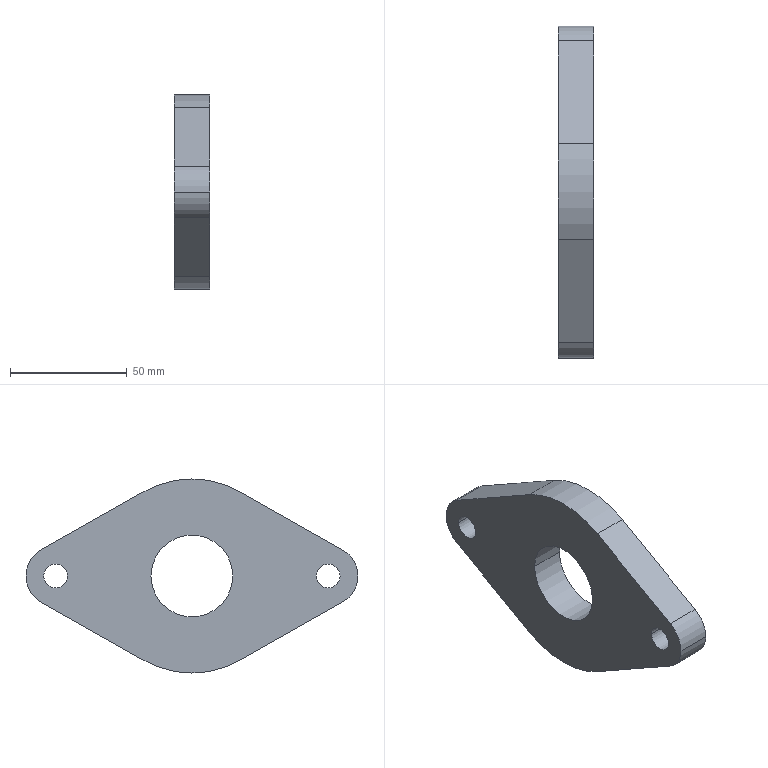Component | SolidWorks | BearingBasePlate-1 | 1 solid | 17 faces | box 15 x 142 x 83 mm | volume 97380 mm3 | cylinder 11 | plane 6 | commonest cylinder face diameters 10.2 x4 25.5 x3 35 x2 83 x2
build123d program:
from build123d import *

# Parameters (mm, degrees)
SKETCH1_R           = 17.5
BOSS_EXTRUDE1_DEPTH = 15
M12_TAPPED_HOLE1_D  = 10.2


with BuildPart() as part:
    # Sketch1 → Boss-Extrude1 (new body)
    with BuildSketch(Plane.XY):
        with BuildLine():
            Line((-20.483, 36.093), (-64.543, 11.089))
            ThreePointArc((-64.543, 11.089), (-71, 0), (-64.543, -11.089))
            Line((-64.543, -11.089), (-20.483, -36.093))
            ThreePointArc((-20.483, -36.093), (0, -41.5), (20.483, -36.093))
            Line((20.483, -36.093), (64.543, -11.089))
            ThreePointArc((64.543, -11.089), (71, 0), (64.543, 11.089))
            Line((64.543, 11.089), (20.483, 36.093))
            ThreePointArc((20.483, 36.093), (0, 41.5), (-20.483, 36.093))
        make_face()
        Circle(SKETCH1_R, mode=Mode.SUBTRACT)
    extrude(amount=BOSS_EXTRUDE1_DEPTH)

    # M12 Tapped Hole1 (through all)
    with Locations(Plane(origin=(0, 0, 0), x_dir=(-1, 0, 0), z_dir=(0, 0, -1))):
        with Locations((-58.25, 0), (58.25, 0)):
            Hole(M12_TAPPED_HOLE1_D / 2)


solid = part.part

# Placed as in the assembly
solid = solid.moved(Location((409.468, 364.666, 811.399), (90, -90, 0)))
STEP:
#1=CARTESIAN_POINT('',(15.53,16.851,31.945));
#2=VERTEX_POINT('',#1);
#3=CARTESIAN_POINT('',(15.53,16.449,31.945));
#4=VERTEX_POINT('',#3);
#5=CARTESIAN_POINT('',(15.53,16.65,31.945));
#6=DIRECTION('',(1.,0.,-0.));
#7=DIRECTION('',(0.,-1.,0.));
#8=AXIS2_PLACEMENT_3D('',#5,#6,#7);
#9=CIRCLE('',#8,0.2008);
#10=EDGE_CURVE('',#2,#4,#9,.T.);
#11=ORIENTED_EDGE('',*,*,#10,.F.);
#12=CARTESIAN_POINT('',(16.121,16.851,31.945));
#13=VERTEX_POINT('',#12);
#14=CARTESIAN_POINT('',(16.121,16.851,31.945));
#15=DIRECTION('',(1.,0.,-0.));
#16=VECTOR('',#15,39.37);
#17=LINE('',#14,#16);
#18=EDGE_CURVE('',#2,#13,#17,.T.);
#19=ORIENTED_EDGE('',*,*,#18,.T.);
#20=CARTESIAN_POINT('',(16.121,16.449,31.945));
#21=VERTEX_POINT('',#20);
#22=CARTESIAN_POINT('',(16.121,16.65,31.945));
#23=DIRECTION('',(1.,0.,-0.));
#24=DIRECTION('',(0.,-1.,0.));
#25=AXIS2_PLACEMENT_3D('',#22,#23,#24);
#26=CIRCLE('',#25,0.2008);
#27=EDGE_CURVE('',#13,#21,#26,.T.);
#28=ORIENTED_EDGE('',*,*,#27,.T.);
#29=CARTESIAN_POINT('',(16.121,16.449,31.945));
#30=DIRECTION('',(1.,0.,-0.));
#31=VECTOR('',#30,39.37);
#32=LINE('',#29,#31);
#33=EDGE_CURVE('',#4,#21,#32,.T.);
#34=ORIENTED_EDGE('',*,*,#33,.F.);
#35=EDGE_LOOP('',(#11,#19,#28,#34));
#36=FACE_OUTER_BOUND('',#35,.T.);
#37=CARTESIAN_POINT('',(16.121,16.65,31.945));
#38=DIRECTION('',(1.,0.,-0.));
#39=DIRECTION('',(0.,-1.,0.));
#40=AXIS2_PLACEMENT_3D('',#37,#38,#39);
#41=CYLINDRICAL_SURFACE('',#40,0.2008);
#42=ADVANCED_FACE('',(#36),#41,.F.);
#43=CARTESIAN_POINT('',(15.53,12.264,31.945));
#44=VERTEX_POINT('',#43);
#45=CARTESIAN_POINT('',(15.53,11.863,31.945));
#46=VERTEX_POINT('',#45);
#47=CARTESIAN_POINT('',(15.53,12.064,31.945));
#48=DIRECTION('',(1.,0.,-0.));
#49=DIRECTION('',(0.,-1.,0.));
#50=AXIS2_PLACEMENT_3D('',#47,#48,#49);
#51=CIRCLE('',#50,0.2008);
#52=EDGE_CURVE('',#44,#46,#51,.T.);
#53=ORIENTED_EDGE('',*,*,#52,.F.);
#54=CARTESIAN_POINT('',(16.121,12.264,31.945));
#55=VERTEX_POINT('',#54);
#56=CARTESIAN_POINT('',(16.121,12.264,31.945));
#57=DIRECTION('',(1.,0.,-0.));
#58=VECTOR('',#57,39.37);
#59=LINE('',#56,#58);
#60=EDGE_CURVE('',#44,#55,#59,.T.);
#61=ORIENTED_EDGE('',*,*,#60,.T.);
#62=CARTESIAN_POINT('',(16.121,11.863,31.945));
#63=VERTEX_POINT('',#62);
#64=CARTESIAN_POINT('',(16.121,12.064,31.945));
#65=DIRECTION('',(1.,0.,-0.));
#66=DIRECTION('',(0.,-1.,0.));
#67=AXIS2_PLACEMENT_3D('',#64,#65,#66);
#68=CIRCLE('',#67,0.2008);
#69=EDGE_CURVE('',#55,#63,#68,.T.);
#70=ORIENTED_EDGE('',*,*,#69,.T.);
#71=CARTESIAN_POINT('',(16.121,11.863,31.945));
#72=DIRECTION('',(1.,0.,-0.));
#73=VECTOR('',#72,39.37);
#74=LINE('',#71,#73);
#75=EDGE_CURVE('',#46,#63,#74,.T.);
#76=ORIENTED_EDGE('',*,*,#75,.F.);
#77=EDGE_LOOP('',(#53,#61,#70,#76));
#78=FACE_OUTER_BOUND('',#77,.T.);
#79=CARTESIAN_POINT('',(16.121,12.064,31.945));
#80=DIRECTION('',(1.,0.,-0.));
#81=DIRECTION('',(0.,-1.,0.));
#82=AXIS2_PLACEMENT_3D('',#79,#80,#81);
#83=CYLINDRICAL_SURFACE('',#82,0.2008);
#84=ADVANCED_FACE('',(#78),#83,.F.);
#85=CARTESIAN_POINT('',(15.53,13.668,31.945));
#86=VERTEX_POINT('',#85);
#87=CARTESIAN_POINT('',(15.53,15.046,31.945));
#88=VERTEX_POINT('',#87);
#89=CARTESIAN_POINT('',(15.53,14.357,31.945));
#90=DIRECTION('',(-1.,-0.,0.));
#91=DIRECTION('',(0.,1.,0.));
#92=AXIS2_PLACEMENT_3D('',#89,#90,#91);
#93=CIRCLE('',#92,0.689);
#94=EDGE_CURVE('',#86,#88,#93,.T.);
#95=ORIENTED_EDGE('',*,*,#94,.T.);
#96=CARTESIAN_POINT('',(16.121,15.046,31.945));
#97=VERTEX_POINT('',#96);
#98=CARTESIAN_POINT('',(15.53,15.046,31.945));
#99=DIRECTION('',(1.,0.,-0.));
#100=VECTOR('',#99,39.37);
#101=LINE('',#98,#100);
#102=EDGE_CURVE('',#88,#97,#101,.T.);
#103=ORIENTED_EDGE('',*,*,#102,.T.);
#104=CARTESIAN_POINT('',(16.121,13.668,31.945));
#105=VERTEX_POINT('',#104);
#106=CARTESIAN_POINT('',(16.121,14.357,31.945));
#107=DIRECTION('',(-1.,-0.,0.));
#108=DIRECTION('',(0.,1.,0.));
#109=AXIS2_PLACEMENT_3D('',#106,#107,#108);
#110=CIRCLE('',#109,0.689);
#111=EDGE_CURVE('',#105,#97,#110,.T.);
#112=ORIENTED_EDGE('',*,*,#111,.F.);
#113=CARTESIAN_POINT('',(15.53,13.668,31.945));
#114=DIRECTION('',(1.,0.,-0.));
#115=VECTOR('',#114,39.37);
#116=LINE('',#113,#115);
#117=EDGE_CURVE('',#86,#105,#116,.T.);
#118=ORIENTED_EDGE('',*,*,#117,.F.);
#119=EDGE_LOOP('',(#95,#103,#112,#118));
#120=FACE_OUTER_BOUND('',#119,.T.);
#121=CARTESIAN_POINT('',(15.53,14.357,31.945));
#122=DIRECTION('',(1.,0.,-0.));
#123=DIRECTION('',(0.,-1.,0.));
#124=AXIS2_PLACEMENT_3D('',#121,#122,#123);
#125=CYLINDRICAL_SURFACE('',#124,0.689);
#126=ADVANCED_FACE('',(#120),#125,.F.);
#127=CARTESIAN_POINT('',(15.53,11.562,31.945));
#128=VERTEX_POINT('',#127);
#129=CARTESIAN_POINT('',(15.53,11.816,32.381));
#130=VERTEX_POINT('',#129);
#131=CARTESIAN_POINT('',(15.53,12.064,31.945));
#132=DIRECTION('',(-1.,-0.,0.));
#133=DIRECTION('',(0.,1.,0.));
#134=AXIS2_PLACEMENT_3D('',#131,#132,#133);
#135=CIRCLE('',#134,0.502);
#136=EDGE_CURVE('',#128,#130,#135,.T.);
#137=ORIENTED_EDGE('',*,*,#136,.F.);
#138=CARTESIAN_POINT('',(16.121,11.562,31.945));
#139=VERTEX_POINT('',#138);
#140=CARTESIAN_POINT('',(15.53,11.562,31.945));
#141=DIRECTION('',(1.,0.,-0.));
#142=VECTOR('',#141,39.37);
#143=LINE('',#140,#142);
#144=EDGE_CURVE('',#128,#139,#143,.T.);
#145=ORIENTED_EDGE('',*,*,#144,.T.);
#146=CARTESIAN_POINT('',(16.121,11.816,32.381));
#147=VERTEX_POINT('',#146);
#148=CARTESIAN_POINT('',(16.121,12.064,31.945));
#149=DIRECTION('',(-1.,-0.,0.));
#150=DIRECTION('',(0.,1.,0.));
#151=AXIS2_PLACEMENT_3D('',#148,#149,#150);
#152=CIRCLE('',#151,0.502);
#153=EDGE_CURVE('',#139,#147,#152,.T.);
#154=ORIENTED_EDGE('',*,*,#153,.T.);
#155=CARTESIAN_POINT('',(15.53,11.816,32.381));
#156=DIRECTION('',(1.,0.,-0.));
#157=VECTOR('',#156,39.37);
#158=LINE('',#155,#157);
#159=EDGE_CURVE('',#130,#147,#158,.T.);
#160=ORIENTED_EDGE('',*,*,#159,.F.);
#161=EDGE_LOOP('',(#137,#145,#154,#160));
#162=FACE_OUTER_BOUND('',#161,.T.);
#163=CARTESIAN_POINT('',(15.53,12.064,31.945));
#164=DIRECTION('',(1.,0.,-0.));
#165=DIRECTION('',(0.,-1.,0.));
#166=AXIS2_PLACEMENT_3D('',#163,#164,#165);
#167=CYLINDRICAL_SURFACE('',#166,0.502);
#168=ADVANCED_FACE('',(#162),#167,.T.);
#169=CARTESIAN_POINT('',(15.53,16.65,31.945));
#170=DIRECTION('',(1.,0.,-0.));
#171=DIRECTION('',(0.,-1.,0.));
#172=AXIS2_PLACEMENT_3D('',#169,#170,#171);
#173=CIRCLE('',#172,0.2008);
#174=EDGE_CURVE('',#4,#2,#173,.T.);
#175=ORIENTED_EDGE('',*,*,#174,.T.);
#176=ORIENTED_EDGE('',*,*,#10,.T.);
#177=EDGE_LOOP('',(#175,#176));
#178=FACE_BOUND('',#177,.T.);
#179=CARTESIAN_POINT('',(15.53,12.064,31.945));
#180=DIRECTION('',(1.,0.,-0.));
#181=DIRECTION('',(0.,-1.,0.));
#182=AXIS2_PLACEMENT_3D('',#179,#180,#181);
#183=CIRCLE('',#182,0.2008);
#184=EDGE_CURVE('',#46,#44,#183,.T.);
#185=ORIENTED_EDGE('',*,*,#184,.T.);
#186=ORIENTED_EDGE('',*,*,#52,.T.);
#187=EDGE_LOOP('',(#185,#186));
#188=FACE_BOUND('',#187,.T.);
#189=CARTESIAN_POINT('',(15.53,15.163,30.524));
#190=VERTEX_POINT('',#189);
#191=CARTESIAN_POINT('',(15.53,13.551,30.524));
#192=VERTEX_POINT('',#191);
#193=CARTESIAN_POINT('',(15.53,14.357,31.945));
#194=DIRECTION('',(-1.,-0.,0.));
#195=DIRECTION('',(0.,1.,0.));
#196=AXIS2_PLACEMENT_3D('',#193,#194,#195);
#197=CIRCLE('',#196,1.634);
#198=EDGE_CURVE('',#190,#192,#197,.T.);
#199=ORIENTED_EDGE('',*,*,#198,.T.);
#200=CARTESIAN_POINT('',(15.53,11.816,31.508));
#201=VERTEX_POINT('',#200);
#202=CARTESIAN_POINT('',(15.53,13.551,30.524));
#203=DIRECTION('',(0.,-0.8697,0.4936));
#204=VECTOR('',#203,39.37);
#205=LINE('',#202,#204);
#206=EDGE_CURVE('',#192,#201,#205,.T.);
#207=ORIENTED_EDGE('',*,*,#206,.T.);
#208=CARTESIAN_POINT('',(15.53,12.064,31.945));
#209=DIRECTION('',(-1.,-0.,0.));
#210=DIRECTION('',(0.,1.,0.));
#211=AXIS2_PLACEMENT_3D('',#208,#209,#210);
#212=CIRCLE('',#211,0.502);
#213=EDGE_CURVE('',#201,#128,#212,.T.);
#214=ORIENTED_EDGE('',*,*,#213,.T.);
#215=ORIENTED_EDGE('',*,*,#136,.T.);
#216=CARTESIAN_POINT('',(15.53,13.551,33.366));
#217=VERTEX_POINT('',#216);
#218=CARTESIAN_POINT('',(15.53,11.816,32.381));
#219=DIRECTION('',(0.,0.8697,0.4936));
#220=VECTOR('',#219,39.37);
#221=LINE('',#218,#220);
#222=EDGE_CURVE('',#130,#217,#221,.T.);
#223=ORIENTED_EDGE('',*,*,#222,.T.);
#224=CARTESIAN_POINT('',(15.53,15.163,33.366));
#225=VERTEX_POINT('',#224);
#226=CARTESIAN_POINT('',(15.53,14.357,31.945));
#227=DIRECTION('',(-1.,-0.,0.));
#228=DIRECTION('',(0.,1.,0.));
#229=AXIS2_PLACEMENT_3D('',#226,#227,#228);
#230=CIRCLE('',#229,1.634);
#231=EDGE_CURVE('',#217,#225,#230,.T.);
#232=ORIENTED_EDGE('',*,*,#231,.T.);
#233=CARTESIAN_POINT('',(15.53,16.898,32.381));
#234=VERTEX_POINT('',#233);
#235=CARTESIAN_POINT('',(15.53,15.163,33.366));
#236=DIRECTION('',(-0.,0.8697,-0.4936));
#237=VECTOR('',#236,39.37);
#238=LINE('',#235,#237);
#239=EDGE_CURVE('',#225,#234,#238,.T.);
#240=ORIENTED_EDGE('',*,*,#239,.T.);
#241=CARTESIAN_POINT('',(15.53,16.898,31.508));
#242=VERTEX_POINT('',#241);
#243=CARTESIAN_POINT('',(15.53,16.65,31.945));
#244=DIRECTION('',(-1.,-0.,0.));
#245=DIRECTION('',(0.,1.,0.));
#246=AXIS2_PLACEMENT_3D('',#243,#244,#245);
#247=CIRCLE('',#246,0.502);
#248=EDGE_CURVE('',#234,#242,#247,.T.);
#249=ORIENTED_EDGE('',*,*,#248,.T.);
#250=CARTESIAN_POINT('',(15.53,16.898,31.508));
#251=DIRECTION('',(-0.,-0.8697,-0.4936));
#252=VECTOR('',#251,39.37);
#253=LINE('',#250,#252);
#254=EDGE_CURVE('',#242,#190,#253,.T.);
#255=ORIENTED_EDGE('',*,*,#254,.T.);
#256=EDGE_LOOP('',(#199,#207,#214,#215,#223,#232,#240,#249,#255));
#257=FACE_OUTER_BOUND('',#256,.T.);
#258=ORIENTED_EDGE('',*,*,#94,.F.);
#259=CARTESIAN_POINT('',(15.53,14.357,31.945));
#260=DIRECTION('',(-1.,-0.,0.));
#261=DIRECTION('',(0.,1.,0.));
#262=AXIS2_PLACEMENT_3D('',#259,#260,#261);
#263=CIRCLE('',#262,0.689);
#264=EDGE_CURVE('',#88,#86,#263,.T.);
#265=ORIENTED_EDGE('',*,*,#264,.F.);
#266=EDGE_LOOP('',(#258,#265));
#267=FACE_BOUND('',#266,.T.);
#268=CARTESIAN_POINT('',(15.53,14.357,31.945));
#269=DIRECTION('',(-1.,-0.,0.));
#270=DIRECTION('',(-0.,1.,0.));
#271=AXIS2_PLACEMENT_3D('',#268,#269,#270);
#272=PLANE('',#271);
#273=ADVANCED_FACE('',(#178,#188,#257,#267),#272,.T.);
#274=CARTESIAN_POINT('',(16.121,16.65,31.945));
#275=DIRECTION('',(1.,0.,-0.));
#276=DIRECTION('',(0.,-1.,0.));
#277=AXIS2_PLACEMENT_3D('',#274,#275,#276);
#278=CIRCLE('',#277,0.2008);
#279=EDGE_CURVE('',#21,#13,#278,.T.);
#280=ORIENTED_EDGE('',*,*,#279,.F.);
#281=ORIENTED_EDGE('',*,*,#27,.F.);
#282=EDGE_LOOP('',(#280,#281));
#283=FACE_BOUND('',#282,.T.);
#284=CARTESIAN_POINT('',(16.121,12.064,31.945));
#285=DIRECTION('',(1.,0.,-0.));
#286=DIRECTION('',(0.,-1.,0.));
#287=AXIS2_PLACEMENT_3D('',#284,#285,#286);
#288=CIRCLE('',#287,0.2008);
#289=EDGE_CURVE('',#63,#55,#288,.T.);
#290=ORIENTED_EDGE('',*,*,#289,.F.);
#291=ORIENTED_EDGE('',*,*,#69,.F.);
#292=EDGE_LOOP('',(#290,#291));
#293=FACE_BOUND('',#292,.T.);
#294=CARTESIAN_POINT('',(16.121,15.163,30.524));
#295=VERTEX_POINT('',#294);
#296=CARTESIAN_POINT('',(16.121,13.551,30.524));
#297=VERTEX_POINT('',#296);
#298=CARTESIAN_POINT('',(16.121,14.357,31.945));
#299=DIRECTION('',(-1.,-0.,0.));
#300=DIRECTION('',(0.,1.,0.));
#301=AXIS2_PLACEMENT_3D('',#298,#299,#300);
#302=CIRCLE('',#301,1.634);
#303=EDGE_CURVE('',#295,#297,#302,.T.);
#304=ORIENTED_EDGE('',*,*,#303,.F.);
#305=CARTESIAN_POINT('',(16.121,16.898,31.508));
#306=VERTEX_POINT('',#305);
#307=CARTESIAN_POINT('',(16.121,16.898,31.508));
#308=DIRECTION('',(-0.,-0.8697,-0.4936));
#309=VECTOR('',#308,39.37);
#310=LINE('',#307,#309);
#311=EDGE_CURVE('',#306,#295,#310,.T.);
#312=ORIENTED_EDGE('',*,*,#311,.F.);
#313=CARTESIAN_POINT('',(16.121,16.898,32.381));
#314=VERTEX_POINT('',#313);
#315=CARTESIAN_POINT('',(16.121,16.65,31.945));
#316=DIRECTION('',(-1.,-0.,0.));
#317=DIRECTION('',(0.,1.,0.));
#318=AXIS2_PLACEMENT_3D('',#315,#316,#317);
#319=CIRCLE('',#318,0.502);
#320=EDGE_CURVE('',#314,#306,#319,.T.);
#321=ORIENTED_EDGE('',*,*,#320,.F.);
#322=CARTESIAN_POINT('',(16.121,15.163,33.366));
#323=VERTEX_POINT('',#322);
#324=CARTESIAN_POINT('',(16.121,15.163,33.366));
#325=DIRECTION('',(-0.,0.8697,-0.4936));
#326=VECTOR('',#325,39.37);
#327=LINE('',#324,#326);
#328=EDGE_CURVE('',#323,#314,#327,.T.);
#329=ORIENTED_EDGE('',*,*,#328,.F.);
#330=CARTESIAN_POINT('',(16.121,13.551,33.366));
#331=VERTEX_POINT('',#330);
#332=CARTESIAN_POINT('',(16.121,14.357,31.945));
#333=DIRECTION('',(-1.,-0.,0.));
#334=DIRECTION('',(0.,1.,0.));
#335=AXIS2_PLACEMENT_3D('',#332,#333,#334);
#336=CIRCLE('',#335,1.634);
#337=EDGE_CURVE('',#331,#323,#336,.T.);
#338=ORIENTED_EDGE('',*,*,#337,.F.);
#339=CARTESIAN_POINT('',(16.121,11.816,32.381));
#340=DIRECTION('',(0.,0.8697,0.4936));
#341=VECTOR('',#340,39.37);
#342=LINE('',#339,#341);
#343=EDGE_CURVE('',#147,#331,#342,.T.);
#344=ORIENTED_EDGE('',*,*,#343,.F.);
#345=ORIENTED_EDGE('',*,*,#153,.F.);
#346=CARTESIAN_POINT('',(16.121,11.816,31.508));
#347=VERTEX_POINT('',#346);
#348=CARTESIAN_POINT('',(16.121,12.064,31.945));
#349=DIRECTION('',(-1.,-0.,0.));
#350=DIRECTION('',(0.,1.,0.));
#351=AXIS2_PLACEMENT_3D('',#348,#349,#350);
#352=CIRCLE('',#351,0.502);
#353=EDGE_CURVE('',#347,#139,#352,.T.);
#354=ORIENTED_EDGE('',*,*,#353,.F.);
#355=CARTESIAN_POINT('',(16.121,13.551,30.524));
#356=DIRECTION('',(0.,-0.8697,0.4936));
#357=VECTOR('',#356,39.37);
#358=LINE('',#355,#357);
#359=EDGE_CURVE('',#297,#347,#358,.T.);
#360=ORIENTED_EDGE('',*,*,#359,.F.);
#361=EDGE_LOOP('',(#304,#312,#321,#329,#338,#344,#345,#354,#360));
#362=FACE_OUTER_BOUND('',#361,.T.);
#363=ORIENTED_EDGE('',*,*,#111,.T.);
#364=CARTESIAN_POINT('',(16.121,14.357,31.945));
#365=DIRECTION('',(-1.,-0.,0.));
#366=DIRECTION('',(0.,1.,0.));
#367=AXIS2_PLACEMENT_3D('',#364,#365,#366);
#368=CIRCLE('',#367,0.689);
#369=EDGE_CURVE('',#97,#105,#368,.T.);
#370=ORIENTED_EDGE('',*,*,#369,.T.);
#371=EDGE_LOOP('',(#363,#370));
#372=FACE_BOUND('',#371,.T.);
#373=CARTESIAN_POINT('',(16.121,14.357,31.945));
#374=DIRECTION('',(-1.,-0.,0.));
#375=DIRECTION('',(-0.,1.,0.));
#376=AXIS2_PLACEMENT_3D('',#373,#374,#375);
#377=PLANE('',#376);
#378=ADVANCED_FACE('',(#283,#293,#362,#372),#377,.F.);
#379=ORIENTED_EDGE('',*,*,#303,.T.);
#380=CARTESIAN_POINT('',(15.53,13.551,30.524));
#381=DIRECTION('',(1.,0.,-0.));
#382=VECTOR('',#381,39.37);
#383=LINE('',#380,#382);
#384=EDGE_CURVE('',#192,#297,#383,.T.);
#385=ORIENTED_EDGE('',*,*,#384,.F.);
#386=ORIENTED_EDGE('',*,*,#198,.F.);
#387=CARTESIAN_POINT('',(15.53,15.163,30.524));
#388=DIRECTION('',(1.,0.,-0.));
#389=VECTOR('',#388,39.37);
#390=LINE('',#387,#389);
#391=EDGE_CURVE('',#190,#295,#390,.T.);
#392=ORIENTED_EDGE('',*,*,#391,.T.);
#393=EDGE_LOOP('',(#379,#385,#386,#392));
#394=FACE_OUTER_BOUND('',#393,.T.);
#395=CARTESIAN_POINT('',(15.53,14.357,31.945));
#396=DIRECTION('',(1.,0.,-0.));
#397=DIRECTION('',(0.,-1.,0.));
#398=AXIS2_PLACEMENT_3D('',#395,#396,#397);
#399=CYLINDRICAL_SURFACE('',#398,1.634);
#400=ADVANCED_FACE('',(#394),#399,.T.);
#401=ORIENTED_EDGE('',*,*,#359,.T.);
#402=CARTESIAN_POINT('',(15.53,11.816,31.508));
#403=DIRECTION('',(1.,0.,-0.));
#404=VECTOR('',#403,39.37);
#405=LINE('',#402,#404);
#406=EDGE_CURVE('',#201,#347,#405,.T.);
#407=ORIENTED_EDGE('',*,*,#406,.F.);
#408=ORIENTED_EDGE('',*,*,#206,.F.);
#409=ORIENTED_EDGE('',*,*,#384,.T.);
#410=EDGE_LOOP('',(#401,#407,#408,#409));
#411=FACE_OUTER_BOUND('',#410,.T.);
#412=CARTESIAN_POINT('',(15.53,13.551,30.524));
#413=DIRECTION('',(0.,0.4936,0.8697));
#414=DIRECTION('',(-0.,0.8697,-0.4936));
#415=AXIS2_PLACEMENT_3D('',#412,#413,#414);
#416=PLANE('',#415);
#417=ADVANCED_FACE('',(#411),#416,.F.);
#418=ORIENTED_EDGE('',*,*,#144,.F.);
#419=ORIENTED_EDGE('',*,*,#213,.F.);
#420=ORIENTED_EDGE('',*,*,#406,.T.);
#421=ORIENTED_EDGE('',*,*,#353,.T.);
#422=EDGE_LOOP('',(#418,#419,#420,#421));
#423=FACE_OUTER_BOUND('',#422,.T.);
#424=CARTESIAN_POINT('',(15.53,12.064,31.945));
#425=DIRECTION('',(1.,0.,-0.));
#426=DIRECTION('',(0.,-1.,0.));
#427=AXIS2_PLACEMENT_3D('',#424,#425,#426);
#428=CYLINDRICAL_SURFACE('',#427,0.502);
#429=ADVANCED_FACE('',(#423),#428,.T.);
#430=ORIENTED_EDGE('',*,*,#343,.T.);
#431=CARTESIAN_POINT('',(15.53,13.551,33.366));
#432=DIRECTION('',(1.,0.,-0.));
#433=VECTOR('',#432,39.37);
#434=LINE('',#431,#433);
#435=EDGE_CURVE('',#217,#331,#434,.T.);
#436=ORIENTED_EDGE('',*,*,#435,.F.);
#437=ORIENTED_EDGE('',*,*,#222,.F.);
#438=ORIENTED_EDGE('',*,*,#159,.T.);
#439=EDGE_LOOP('',(#430,#436,#437,#438));
#440=FACE_OUTER_BOUND('',#439,.T.);
#441=CARTESIAN_POINT('',(15.53,11.816,32.381));
#442=DIRECTION('',(-0.,0.4936,-0.8697));
#443=DIRECTION('',(-0.,-0.8697,-0.4936));
#444=AXIS2_PLACEMENT_3D('',#441,#442,#443);
#445=PLANE('',#444);
#446=ADVANCED_FACE('',(#440),#445,.F.);
#447=ORIENTED_EDGE('',*,*,#337,.T.);
#448=CARTESIAN_POINT('',(15.53,15.163,33.366));
#449=DIRECTION('',(1.,0.,-0.));
#450=VECTOR('',#449,39.37);
#451=LINE('',#448,#450);
#452=EDGE_CURVE('',#225,#323,#451,.T.);
#453=ORIENTED_EDGE('',*,*,#452,.F.);
#454=ORIENTED_EDGE('',*,*,#231,.F.);
#455=ORIENTED_EDGE('',*,*,#435,.T.);
#456=EDGE_LOOP('',(#447,#453,#454,#455));
#457=FACE_OUTER_BOUND('',#456,.T.);
#458=CARTESIAN_POINT('',(15.53,14.357,31.945));
#459=DIRECTION('',(1.,0.,-0.));
#460=DIRECTION('',(0.,-1.,0.));
#461=AXIS2_PLACEMENT_3D('',#458,#459,#460);
#462=CYLINDRICAL_SURFACE('',#461,1.634);
#463=ADVANCED_FACE('',(#457),#462,.T.);
#464=ORIENTED_EDGE('',*,*,#328,.T.);
#465=CARTESIAN_POINT('',(15.53,16.898,32.381));
#466=DIRECTION('',(1.,0.,-0.));
#467=VECTOR('',#466,39.37);
#468=LINE('',#465,#467);
#469=EDGE_CURVE('',#234,#314,#468,.T.);
#470=ORIENTED_EDGE('',*,*,#469,.F.);
#471=ORIENTED_EDGE('',*,*,#239,.F.);
#472=ORIENTED_EDGE('',*,*,#452,.T.);
#473=EDGE_LOOP('',(#464,#470,#471,#472));
#474=FACE_OUTER_BOUND('',#473,.T.);
#475=CARTESIAN_POINT('',(15.53,15.163,33.366));
#476=DIRECTION('',(-0.,-0.4936,-0.8697));
#477=DIRECTION('',(0.,-0.8697,0.4936));
#478=AXIS2_PLACEMENT_3D('',#475,#476,#477);
#479=PLANE('',#478);
#480=ADVANCED_FACE('',(#474),#479,.F.);
#481=ORIENTED_EDGE('',*,*,#320,.T.);
#482=CARTESIAN_POINT('',(15.53,16.898,31.508));
#483=DIRECTION('',(1.,0.,-0.));
#484=VECTOR('',#483,39.37);
#485=LINE('',#482,#484);
#486=EDGE_CURVE('',#242,#306,#485,.T.);
#487=ORIENTED_EDGE('',*,*,#486,.F.);
#488=ORIENTED_EDGE('',*,*,#248,.F.);
#489=ORIENTED_EDGE('',*,*,#469,.T.);
#490=EDGE_LOOP('',(#481,#487,#488,#489));
#491=FACE_OUTER_BOUND('',#490,.T.);
#492=CARTESIAN_POINT('',(15.53,16.65,31.945));
#493=DIRECTION('',(1.,0.,-0.));
#494=DIRECTION('',(0.,-1.,0.));
#495=AXIS2_PLACEMENT_3D('',#492,#493,#494);
#496=CYLINDRICAL_SURFACE('',#495,0.502);
#497=ADVANCED_FACE('',(#491),#496,.T.);
#498=ORIENTED_EDGE('',*,*,#311,.T.);
#499=ORIENTED_EDGE('',*,*,#391,.F.);
#500=ORIENTED_EDGE('',*,*,#254,.F.);
#501=ORIENTED_EDGE('',*,*,#486,.T.);
#502=EDGE_LOOP('',(#498,#499,#500,#501));
#503=FACE_OUTER_BOUND('',#502,.T.);
#504=CARTESIAN_POINT('',(15.53,16.898,31.508));
#505=DIRECTION('',(0.,-0.4936,0.8697));
#506=DIRECTION('',(0.,0.8697,0.4936));
#507=AXIS2_PLACEMENT_3D('',#504,#505,#506);
#508=PLANE('',#507);
#509=ADVANCED_FACE('',(#503),#508,.F.);
#510=ORIENTED_EDGE('',*,*,#102,.F.);
#511=ORIENTED_EDGE('',*,*,#264,.T.);
#512=ORIENTED_EDGE('',*,*,#117,.T.);
#513=ORIENTED_EDGE('',*,*,#369,.F.);
#514=EDGE_LOOP('',(#510,#511,#512,#513));
#515=FACE_OUTER_BOUND('',#514,.T.);
#516=CARTESIAN_POINT('',(15.53,14.357,31.945));
#517=DIRECTION('',(1.,0.,-0.));
#518=DIRECTION('',(0.,-1.,0.));
#519=AXIS2_PLACEMENT_3D('',#516,#517,#518);
#520=CYLINDRICAL_SURFACE('',#519,0.689);
#521=ADVANCED_FACE('',(#515),#520,.F.);
#522=ORIENTED_EDGE('',*,*,#60,.F.);
#523=ORIENTED_EDGE('',*,*,#184,.F.);
#524=ORIENTED_EDGE('',*,*,#75,.T.);
#525=ORIENTED_EDGE('',*,*,#289,.T.);
#526=EDGE_LOOP('',(#522,#523,#524,#525));
#527=FACE_OUTER_BOUND('',#526,.T.);
#528=CARTESIAN_POINT('',(16.121,12.064,31.945));
#529=DIRECTION('',(1.,0.,-0.));
#530=DIRECTION('',(0.,-1.,0.));
#531=AXIS2_PLACEMENT_3D('',#528,#529,#530);
#532=CYLINDRICAL_SURFACE('',#531,0.2008);
#533=ADVANCED_FACE('',(#527),#532,.F.);
#534=ORIENTED_EDGE('',*,*,#18,.F.);
#535=ORIENTED_EDGE('',*,*,#174,.F.);
#536=ORIENTED_EDGE('',*,*,#33,.T.);
#537=ORIENTED_EDGE('',*,*,#279,.T.);
#538=EDGE_LOOP('',(#534,#535,#536,#537));
#539=FACE_OUTER_BOUND('',#538,.T.);
#540=CARTESIAN_POINT('',(16.121,16.65,31.945));
#541=DIRECTION('',(1.,0.,-0.));
#542=DIRECTION('',(0.,-1.,0.));
#543=AXIS2_PLACEMENT_3D('',#540,#541,#542);
#544=CYLINDRICAL_SURFACE('',#543,0.2008);
#545=ADVANCED_FACE('',(#539),#544,.F.);
#546=CLOSED_SHELL('',(#42,#84,#126,#168,#273,#378,#400,#417,#429,#446,#463,#480,#497,#509,#521,#533,#545));
#547=MANIFOLD_SOLID_BREP('',#546);
#548=CARTESIAN_POINT('',(0.,0.,0.));
#549=DIRECTION('',(0.,0.,1.));
#550=DIRECTION('',(1.,0.,0.));
#551=AXIS2_PLACEMENT_3D('',#548,#549,#550);
#552=(LENGTH_UNIT()NAMED_UNIT(*)SI_UNIT($,.METRE.));
#553=LENGTH_MEASURE_WITH_UNIT(LENGTH_MEASURE(0.0254),#552);
#554=DIMENSIONAL_EXPONENTS(1.,0.,0.,0.,0.,0.,0.);
#555=(CONVERSION_BASED_UNIT('',#553)LENGTH_UNIT()NAMED_UNIT(#554));
#556=UNCERTAINTY_MEASURE_WITH_UNIT(LENGTH_MEASURE(0.00001),#555,'','');
#557=(NAMED_UNIT(*)PLANE_ANGLE_UNIT()SI_UNIT($,.RADIAN.));
#558=(NAMED_UNIT(*)SI_UNIT($,.STERADIAN.)SOLID_ANGLE_UNIT());
#559=(GEOMETRIC_REPRESENTATION_CONTEXT(3)GLOBAL_UNCERTAINTY_ASSIGNED_CONTEXT((#556))GLOBAL_UNIT_ASSIGNED_CONTEXT((#555,#557,#558))REPRESENTATION_CONTEXT('',''));
#560=ADVANCED_BREP_SHAPE_REPRESENTATION('',(#547,#551),#559);
#561=COLOUR_RGB('',0.7922,0.8196,0.9333);
#562=FILL_AREA_STYLE_COLOUR('',#561);
#563=FILL_AREA_STYLE('',(#562));
#564=SURFACE_STYLE_FILL_AREA(#563);
#565=SURFACE_SIDE_STYLE('',(#564));
#566=SURFACE_STYLE_USAGE(.BOTH.,#565);
#567=PRESENTATION_STYLE_ASSIGNMENT((#566));
#568=STYLED_ITEM('',(#567),#547);
#569=(LENGTH_UNIT()NAMED_UNIT(*)SI_UNIT($,.METRE.));
#570=LENGTH_MEASURE_WITH_UNIT(LENGTH_MEASURE(0.0254),#569);
#571=DIMENSIONAL_EXPONENTS(1.,0.,0.,0.,0.,0.,0.);
#572=(CONVERSION_BASED_UNIT('',#570)LENGTH_UNIT()NAMED_UNIT(#571));
#573=UNCERTAINTY_MEASURE_WITH_UNIT(LENGTH_MEASURE(0.00001),#572,'','');
#574=(NAMED_UNIT(*)PLANE_ANGLE_UNIT()SI_UNIT($,.RADIAN.));
#575=(NAMED_UNIT(*)SI_UNIT($,.STERADIAN.)SOLID_ANGLE_UNIT());
#576=(GEOMETRIC_REPRESENTATION_CONTEXT(3)GLOBAL_UNCERTAINTY_ASSIGNED_CONTEXT((#573))GLOBAL_UNIT_ASSIGNED_CONTEXT((#572,#574,#575))REPRESENTATION_CONTEXT('',''));
#577=MECHANICAL_DESIGN_GEOMETRIC_PRESENTATION_REPRESENTATION('',(#568),#576);
#578=PRESENTATION_LAYER_ASSIGNMENT('','',(#568));